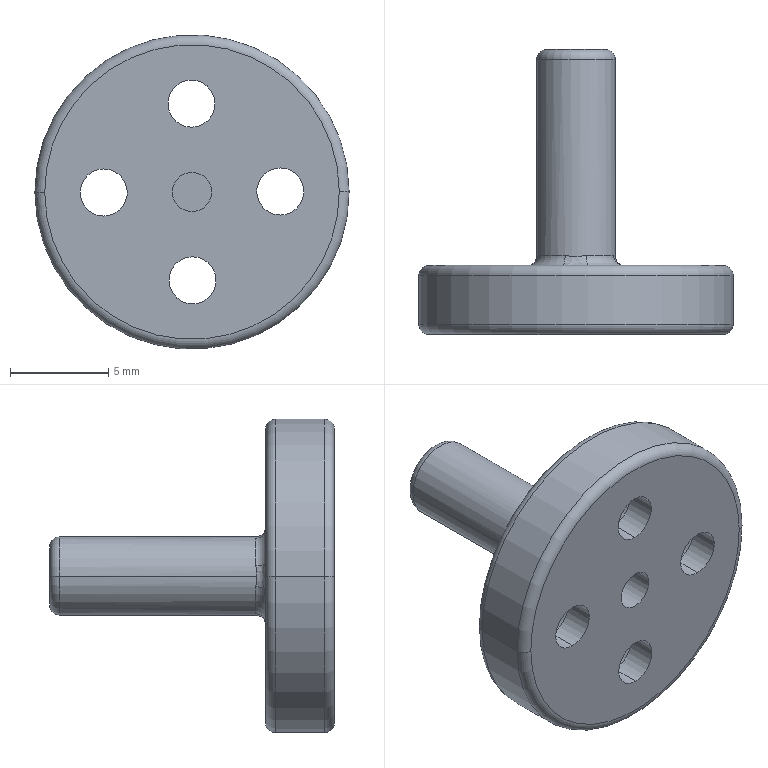Component | SolidWorks | 5.Spinner-1 | 1 solid | 44 faces | box 16 x 14.5 x 16 mm | volume 675 mm3 | cylinder 22 | torus 10 | plane 8 | spline 4 | commonest cylinder face diameters 4.4 x8 2.4 x8 2 x2 4 x2 16 x2